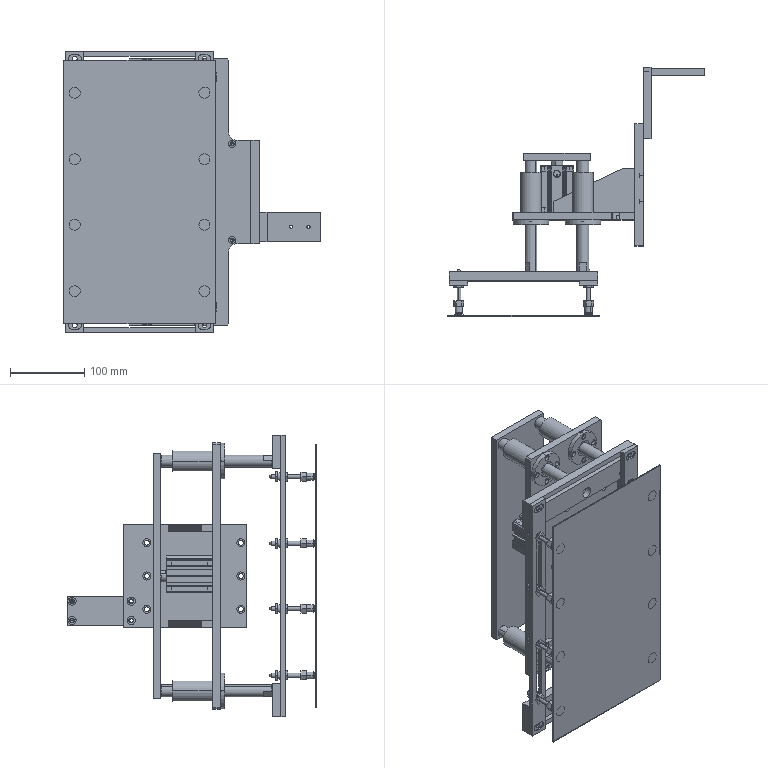Assembly | SolidWorks | mm | 30 component files | 30 solids | 1263 faces | box 346.5 x 335.9 x 380 mm | volume 1913881 mm3 | cylinder 546 | plane 505 | cone 168 | torus 32 | spline 12 | commonest cylinder face diameters 10 x40 0.4 x36 3.3 x32 4.5 x32 7.5 x32 6 x32 11 x28 6.6 x28
Bill of materials:
SL021-102-4065.SL4PRT | 4 | Bearing Steel | Long, slender cylindrical rod with a small axial hole at one end and a short flat on the outside next to that end.
SL021-102-4066.SL4PRT | 1 | AL6061 | Flat rectangular plate of even thickness with many round through holes spread around its edges and in the interior.
SL021-102-4067.SL4PRT | 2 | AL6061 | Flat plate of even thickness with a trapezoid outline (one sloped edge), with holes drilled into its narrow side edges.
SL021-102-4073.SL4PRT | 1 | AL6061 | Rectangular block or thick plate with four round through holes near its corners. The two holes at one end look larger than the two at the other.
SL021-102-4074.SL4PRT | 1 | AL6061 | Rectangular block with two small round through holes in a row on one large face, set off-center toward one end.
SL021-102-4096.SL4PRT | 1 | AL6061 | Long rectangular bar with one long slot with rounded ends running along one edge, and two round through holes near the opposite edge, toward one end.
SL021-102-4097.SL4PRT | 1 | AL6061 | Long rectangular bar with one long slot with rounded ends near one long edge, and two round through holes near the opposite edge, toward one end.
SL021-102-4098.SL4PRT | 2 | AL6061 | Thin, long, narrow strip with two long slots with rounded ends along its center line and a small round hole near each end.
SL021-102-4099.SL4PRT | 1 | AL6061 | Flat plate shaped like a rectangle with a tab sticking out from one long side. Rounded notches sit where the tab meets the plate. Four large round holes, each ringed by four small holes, are near the corners, with more small holes in the middle and on the tab.
SL021-102-4100.SL4PRT | 1 | AL6061 | Thin flat rectangular plate with four small round holes near the corners and one small hole in the center.
SL021-113Q32x30S (1)-2.sl4prt | 1 |  | Stepped round pin: a large-diameter head with grooves around it and a wider collar, then a smaller straight shaft with a short flat near its free end.
SL021-113Q32x30S (2)-2.sl4prt | 1 |  | Prism-shaped body made by extruding a near-square cross-section, with a large central round bore, four smaller holes running the full length near the corners, and slots running lengthwise on its sides. One side has a raised pad with two round holes.
SL021-1LGP-15.6.SL4PRT | 1 | AL6061 | Flat rectangular plate or sheet with no visible thickness and no holes or other features.
SL021-1RoundFlangeExtendedType-416.SL4PRT | 4 | Q235 | Flanged cylindrical sleeve: a long round tube with a round flange at one end. The flange has four evenly spaced holes around a central through-bore.
SL021-1SuctionCup.SL4PRT | 8 | AL6061 | Stepped round shaft with a wide flared, conical head at one end and a chamfered tip at the other. Three hexagonal features sit along the shaft.
Mates:
1. coincident | SL021-102-4097.SL4PRT-1 face at (-136.163, -102.499, 16.122) dir (0, -1, 0) | SL021-102-4098.SL4PRT-5 face at (-223.663, -102.499, -151.378) dir (0, 1, 0)
2. coincident | SL021-102-4098.SL4PRT-5 face at (-223.663, -102.499, -151.378) dir (0, 1, 0) | SL021-102-4098.SL4PRT-6 face at (-48.663, -102.499, -151.378) dir (0, 1, 0)
3. coincident | SL021-102-4098.SL4PRT-5 face at (-236.163, -102.499, 38.622) dir (0, 0, 1) | SL021-102-4098.SL4PRT-6 face at (-61.163, -102.499, 38.622) dir (0, 0, 1)
4. coincident | SL021-102-4097.SL4PRT-1 face at (-36.163, -90.499, 38.622) dir (1, 0, 0) | SL021-102-4096.SL4PRT-1 face at (-36.163, -102.499, -341.378) dir (1, 0, 0)
5. coincident | SL021-102-4065.SL4PRT-5 face at (-126.163, 59.501, -306.378) dir (0, 1, 0) | SL021-102-4100.SL4PRT-1 face at (-91.163, 59.501, -151.378) dir (0, -1, 0)
6. concentric | SL021-102-4065.SL4PRT-5 face at (-126.163, 59.501, -306.378) dir (0, -1, 0) r 8 | SL021-102-4099.SL4PRT-1 face at (-126.163, -10.499, -306.378) dir (0, -1, 0) r 14.05
7. coincident | SL021-102-4099.SL4PRT-1 face at (-83.663, -10.499, -151.378) dir (0, 1, 0) | SL021-113Q32x30S-2.SL41SM-1/SL021-113Q32x30S (2)-2.sl4prt-1 face at (-91.163, -10.499, -151.378) dir (0, -1, 0)
8. width | SL021-102-4099.SL4PRT-1 face at (-16.163, -20.499, -331.378) dir (0, 0, -1) | SL021-102-4099.SL4PRT-1 face at (-16.163, -20.499, 28.622) dir (0, 0, 1) | SL021-113Q32x30S-2.SL41SM-1/SL021-113Q32x30S (2)-2.sl4prt-1 face at (-104.663, 52.501, -173.878) dir (0, 0, -1) | SL021-113Q32x30S-2.SL41SM-1/SL021-113Q32x30S (2)-2.sl4prt-1 face at (-111.663, 52.501, -128.878) dir (0, 0, 1)
9. coincident | SL021-102-4100.SL4PRT-1 face at (-91.163, 59.501, -151.378) dir (0, -1, 0) | SL021-113Q32x30S-2.SL41SM-1/SL021-113Q32x30S (1)-2.sl4prt-1 face at (-88.197, 59.501, -148.885) dir (0, 1, 0)
10. coincident | SL021-102-4098.SL4PRT-6 face at (-48.663, -108.499, -151.378) dir (0, -1, 0) | SL021-1SuctionCup.SL4PRT-1 face at (-48.663, -108.499, -17.378) dir (0, 1, 0)
11. concentric | SL021-102-4098.SL4PRT-6 face at (-48.663, -108.499, -17.378) dir (0, 1, 0) r 5.25 | SL021-1SuctionCup.SL4PRT-1 face at (-48.663, -129.499, -17.378) dir (0, 1, 0) r 3
12. coincident | SL021-1SuctionCup.SL4PRT-1 face at (-48.663, -149.499, -17.378) dir (0, -1, 0) | SL021-1SuctionCup.SL4PRT-2 face at (-223.663, -149.499, -17.378) dir (0, -1, 0)
13. coincident | SL021-1SuctionCup.SL4PRT-2 face at (-223.663, -149.499, -17.378) dir (0, -1, 0) | SL021-1SuctionCup.SL4PRT-3 face at (-48.663, -149.499, -285.378) dir (0, -1, 0)
14. coincident | SL021-1SuctionCup.SL4PRT-3 face at (-48.663, -149.499, -285.378) dir (0, -1, 0) | SL021-1SuctionCup.SL4PRT-4 face at (-223.663, -149.499, -285.378) dir (0, -1, 0)
15. coincident | SL021-1SuctionCup.SL4PRT-4 face at (-223.663, -149.499, -285.378) dir (0, -1, 0) | SL021-1SuctionCup.SL4PRT-5 face at (-48.663, -149.499, -195.378) dir (0, -1, 0)
16. coincident | SL021-1SuctionCup.SL4PRT-5 face at (-48.663, -149.499, -195.378) dir (0, -1, 0) | SL021-1SuctionCup.SL4PRT-6 face at (-48.663, -149.499, -107.378) dir (0, -1, 0)
17. coincident | SL021-1SuctionCup.SL4PRT-6 face at (-48.663, -149.499, -107.378) dir (0, -1, 0) | SL021-1SuctionCup.SL4PRT-7 face at (-223.663, -149.499, -107.378) dir (0, -1, 0)
18. coincident | SL021-1SuctionCup.SL4PRT-7 face at (-223.663, -149.499, -107.378) dir (0, -1, 0) | SL021-1SuctionCup.SL4PRT-8 face at (-223.663, -149.499, -195.378) dir (0, -1, 0)
19. concentric | SL021-102-4098.SL4PRT-5 face at (-223.663, -108.499, -17.378) dir (0, 1, 0) r 5.25 | SL021-1SuctionCup.SL4PRT-2 face at (-223.663, -98.499, -17.378) dir (0, -1, 0) r 5
20. concentric | SL021-102-4098.SL4PRT-6 face at (-48.663, -108.499, -285.378) dir (0, 1, 0) r 5.25 | SL021-1SuctionCup.SL4PRT-3 face at (-48.663, -129.499, -285.378) dir (0, 1, 0) r 3
21. concentric | SL021-102-4098.SL4PRT-5 face at (-223.663, -108.499, -285.378) dir (0, 1, 0) r 5.25 | SL021-1SuctionCup.SL4PRT-4 face at (-223.663, -129.499, -285.378) dir (0, 1, 0) r 3
22. concentric | SL021-102-4098.SL4PRT-6 face at (-48.663, -108.499, -195.378) dir (0, 1, 0) r 5.25 | SL021-1SuctionCup.SL4PRT-5 face at (-48.663, -129.499, -195.378) dir (0, 1, 0) r 3
23. concentric | SL021-102-4098.SL4PRT-6 face at (-48.663, -108.499, -107.378) dir (0, 1, 0) r 5.25 | SL021-1SuctionCup.SL4PRT-6 face at (-48.663, -129.499, -107.378) dir (0, 1, 0) r 3
24. concentric | SL021-102-4098.SL4PRT-5 face at (-223.663, -108.499, -107.378) dir (0, 1, 0) r 5.25 | SL021-1SuctionCup.SL4PRT-7 face at (-223.663, -87.499, -107.378) dir (0, -1, 0) r 3
25. concentric | SL021-102-4098.SL4PRT-5 face at (-223.663, -108.499, -195.378) dir (0, 1, 0) r 5.25 | SL021-1SuctionCup.SL4PRT-8 face at (-223.663, -129.499, -195.378) dir (0, 1, 0) r 3
26. coincident | SL021-102-4099.SL4PRT-1 face at (13.837, -20.499, -81.378) dir (0, 0, 1) | SL021-102-4066.SL4PRT-1 face at (25.837, -55.499, -81.378) dir (0, 0, 1)
27. coincident | SL021-102-4067.SL4PRT-1 face at (13.837, 49.501, -91.378) dir (0, 1, 0) | SL021-102-4067.SL4PRT-2 face at (13.837, 49.501, -221.378) dir (0, 1, 0)
28. coincident | SL021-102-4067.SL4PRT-1 face at (13.837, -10.499, -91.378) dir (1, 0, 0) | SL021-102-4067.SL4PRT-2 face at (13.837, -10.499, -221.378) dir (1, 0, 0)
29. coincident | SL021-102-4099.SL4PRT-1 face at (-83.663, -10.499, -151.378) dir (0, 1, 0) | SL021-102-4067.SL4PRT-1 face at (-96.163, -10.499, -91.378) dir (0, -1, 0)
30. coincident | SL021-102-4066.SL4PRT-1 face at (13.837, 27.001, -151.378) dir (-1, 0, 0) | SL021-102-4067.SL4PRT-1 face at (13.837, -10.499, -91.378) dir (1, 0, 0)
31. coincident | SL021-102-4066.SL4PRT-1 face at (25.837, -55.499, -81.378) dir (0, 0, 1) | SL021-102-4067.SL4PRT-1 face at (13.837, -10.499, -81.378) dir (0, 0, 1)
32. coincident | SL021-102-4066.SL4PRT-1 face at (25.837, -55.499, -221.378) dir (0, 0, -1) | SL021-102-4067.SL4PRT-2 face at (13.837, -10.499, -221.378) dir (0, 0, -1)
33. coincident | SL021-102-4073.SL4PRT-1 face at (35.837, 137.501, -198.378) dir (1, 0, 0) | SL021-102-4074.SL4PRT-1 face at (35.837, 184.501, -218.378) dir (-1, 0, 0)
34. concentric | SL021-102-4073.SL4PRT-1 face at (25.837, 179.501, -185.378) dir (-1, 0, 0) r 5.5 | SL021-102-4074.SL4PRT-1 face at (35.837, 179.501, -185.378) dir (-1, 0, 0) r 2.5
35. parallel | SL021-102-4073.SL4PRT-1 face at (25.837, 185.501, -218.378) dir (0, 1, 0) | SL021-102-4074.SL4PRT-1 face at (71.837, 184.501, -198.378) dir (0, 1, 0)
36. coincident | SL021-102-4066.SL4PRT-1 face at (25.837, 27.001, -151.378) dir (1, 0, 0) | SL021-102-4073.SL4PRT-1 face at (25.837, 137.501, -198.378) dir (-1, 0, 0)
37. concentric | SL021-102-4066.SL4PRT-1 face at (13.837, 99.501, -211.378) dir (-1, 0, 0) r 3.3 | SL021-102-4073.SL4PRT-1 face at (25.837, 99.501, -211.378) dir (-1, 0, 0) r 2.5
38. concentric | SL021-102-4066.SL4PRT-1 face at (13.837, 99.501, -185.378) dir (-1, 0, 0) r 3.3 | SL021-102-4073.SL4PRT-1 face at (25.837, 99.501, -185.378) dir (-1, 0, 0) r 2.5
39. coincident | SL021-102-4098.SL4PRT-6 face at (-36.163, -102.499, -341.378) dir (1, 0, 0) | SL021-102-4096.SL4PRT-1 face at (-36.163, -102.499, -341.378) dir (1, 0, 0)
40. coincident | SL021-102-4098.SL4PRT-5 face at (-236.163, -102.499, -341.378) dir (-1, 0, 0) | SL021-102-4096.SL4PRT-1 face at (-236.163, -102.499, -341.378) dir (-1, 0, 0)
41. concentric | SL021-102-4099.SL4PRT-1 face at (-126.163, -10.499, -306.378) dir (0, -1, 0) r 14.05 | SL021-1RoundFlangeExtendedType-416.SL4PRT-1 face at (-126.163, 43.501, -306.378) dir (0, 1, 0) r 14
42. coincident | SL021-102-4099.SL4PRT-1 face at (-83.663, -20.499, -151.378) dir (0, -1, 0) | SL021-1RoundFlangeExtendedType-416.SL4PRT-1 face at (-126.163, -20.499, -318.378) dir (0, 1, 0)
43. parallel | SL021-102-4099.SL4PRT-1 face at (-151.163, -20.499, -331.378) dir (-1, 0, 0) | SL021-1RoundFlangeExtendedType-416.SL4PRT-1 plane at (-126.163, -26.499, -306.378) dir (-1, 0, 0)
44. parallel | SL021-102-4100.SL4PRT-1 face at (-136.163, 59.501, -316.378) dir (-1, 0, 0) | SL021-102-4099.SL4PRT-1 face at (-151.163, -20.499, -331.378) dir (-1, 0, 0)
45. parallel | SL021-102-4097.SL4PRT-1 face at (-236.163, -90.499, -6.378) dir (0, 0, -1) | SL021-102-4099.SL4PRT-1 face at (-16.163, -20.499, 28.622) dir (0, 0, 1)
46. coincident | SL021-102-4097.SL4PRT-1 face at (-236.163, -90.499, 38.622) dir (0, 0, 1) | SL021-102-4098.SL4PRT-5 face at (-236.163, -102.499, 38.622) dir (0, 0, 1)
47. coincident | SL021-102-4099.SL4PRT-1 face at (-83.663, -20.499, -151.378) dir (0, -1, 0) | SL021-1RoundFlangeExtendedType-416.SL4PRT-4 face at (-56.163, -20.499, 15.622) dir (0, 1, 0)
48. coincident | SL021-102-4099.SL4PRT-1 face at (-83.663, -20.499, -151.378) dir (0, -1, 0) | SL021-1RoundFlangeExtendedType-416.SL4PRT-3 face at (-56.163, -20.499, -294.378) dir (0, 1, 0)
49. parallel | SL021-102-4099.SL4PRT-1 face at (-151.163, -20.499, -331.378) dir (-1, 0, 0) | SL021-1RoundFlangeExtendedType-416.SL4PRT-3 plane at (-56.163, -26.499, -306.378) dir (1, 0, 0)
50. parallel | SL021-102-4099.SL4PRT-1 face at (-151.163, -20.499, -331.378) dir (-1, 0, 0) | SL021-1RoundFlangeExtendedType-416.SL4PRT-4 plane at (-56.163, -26.499, 3.622) dir (1, 0, 0)
51. concentric | SL021-1RoundFlangeExtendedType-416.SL4PRT-3 face at (-56.163, 43.501, -306.378) dir (0, 1, 0) r 8 | SL021-102-4065.SL4PRT-8 face at (-56.163, 59.501, -306.378) dir (0, -1, 0) r 8
52. concentric | SL021-1RoundFlangeExtendedType-416.SL4PRT-4 face at (-56.163, 43.501, 3.622) dir (0, 1, 0) r 14 | SL021-102-4065.SL4PRT-9 face at (-56.163, 59.501, 3.622) dir (0, -1, 0) r 8
53. coincident | SL021-102-4065.SL4PRT-8 face at (-56.163, 59.501, -306.378) dir (0, 1, 0) | SL021-102-4065.SL4PRT-9 face at (-56.163, 59.501, 3.622) dir (0, 1, 0)
54. coincident | SL021-102-4100.SL4PRT-1 face at (-91.163, 59.501, -151.378) dir (0, -1, 0) | SL021-102-4065.SL4PRT-9 face at (-56.163, 59.501, 3.622) dir (0, 1, 0)
55. concentric | SL021-102-4099.SL4PRT-1 face at (-56.163, -10.499, 3.622) dir (0, -1, 0) r 14.05 | SL021-1RoundFlangeExtendedType-416.SL4PRT-4 face at (-56.163, 43.501, 3.622) dir (0, 1, 0) r 14
56. concentric | SL021-102-4099.SL4PRT-1 face at (-56.163, -10.499, -306.378) dir (0, -1, 0) r 14.05 | SL021-1RoundFlangeExtendedType-416.SL4PRT-3 face at (-56.163, 43.501, -306.378) dir (0, 1, 0) r 14
57. concentric | SL021-102-4065.SL4PRT-5 face at (-126.163, 59.501, -306.378) dir (0, -1, 0) r 8 | SL021-102-4096.SL4PRT-1 face at (-126.163, -102.499, -306.378) dir (0, -1, 0) r 7.5
58. coincident | SL021-102-4097.SL4PRT-1 face at (-136.163, -90.499, 16.122) dir (0, 1, 0) | SL021-102-4096.SL4PRT-1 face at (-136.163, -90.499, -318.878) dir (0, 1, 0)
59. coincident | SL021-102-4097.SL4PRT-1 face at (-136.163, -90.499, 16.122) dir (0, 1, 0) | SL021-102-4065.SL4PRT-5 face at (-126.163, -90.499, -306.378) dir (0, -1, 0)
60. coincident | SL021-1SuctionCup.SL4PRT-2 face at (-223.663, -149.499, -17.378) dir (0, -1, 0) | SL021-1LGP-15.6.SL4PRT-1 face at (-136.163, -149.499, -151.378) dir (0, 1, 0)
61. concentric | SL021-102-4100.SL4PRT-1 face at (-126.163, 59.501, 3.622) dir (0, -1, 0) r 4.25 | SL021-102-4065.SL4PRT-7 face at (-126.163, 59.501, 3.622) dir (0, -1, 0) r 8
62. width | SL021-102-4100.SL4PRT-1 face at (-136.163, 59.501, -316.378) dir (-1, 0, 0) | SL021-102-4100.SL4PRT-1 face at (-46.163, 59.501, -316.378) dir (1, 0, 0) | SL021-113Q32x30S-2.SL41SM-1/SL021-113Q32x30S (2)-2.sl4prt-1 face at (-113.663, 52.501, -137.878) dir (-1, 0, 0) | SL021-113Q32x30S-2.SL41SM-1/SL021-113Q32x30S (2)-2.sl4prt-1 face at (-68.663, 52.501, -130.878) dir (1, 0, 0)
63. width | SL021-102-4096.SL4PRT-1 face at (-236.163, -102.499, -341.378) dir (-1, 0, 0) | SL021-102-4096.SL4PRT-1 face at (-36.163, -102.499, -341.378) dir (1, 0, 0) | SL021-1LGP-15.6.SL4PRT-1 face at (-238.663, -149.499, -328.878) dir (-1, 0, 0) | SL021-1LGP-15.6.SL4PRT-1 face at (-33.663, -149.499, -328.878) dir (1, 0, 0)
64. width | SL021-1LGP-15.6.SL4PRT-1 face at (-238.663, -149.499, -328.878) dir (0, 0, -1) | SL021-1LGP-15.6.SL4PRT-1 face at (-238.663, -149.499, 26.122) dir (0, 0, 1) | SL021-102-4096.SL4PRT-1 face at (-236.163, -102.499, -341.378) dir (0, 0, -1) | SL021-102-4097.SL4PRT-1 face at (-236.163, -90.499, 38.622) dir (0, 0, 1)
65. width | SL021-102-4096.SL4PRT-1 face at (-236.163, -102.499, -341.378) dir (0, 0, -1) | SL021-102-4097.SL4PRT-1 face at (-236.163, -90.499, 38.622) dir (0, 0, 1) | SL021-102-4099.SL4PRT-1 face at (-16.163, -20.499, -331.378) dir (0, 0, -1) | SL021-102-4099.SL4PRT-1 face at (-16.163, -20.499, 28.622) dir (0, 0, 1)
66. coincident | SL021-102-4099.SL4PRT-1 face at (13.837, -15.499, -151.378) dir (1, 0, 0) | SL021-102-4066.SL4PRT-1 face at (13.837, 27.001, -151.378) dir (-1, 0, 0)
67. distance | SL021-102-4099.SL4PRT-1 face at (-83.663, -20.499, -151.378) dir (0, -1, 0) | SL021-102-4066.SL4PRT-1 face at (25.837, 109.501, -81.378) dir (0, 1, 0)
68. concentric | SL021-113Q32x30S (1)-2.sl4prt-1 face at (-3.375, 0, 0) dir (1, 0, 0) r 8 | SL021-113Q32x30S (2)-2.sl4prt-1 face at (34.5, 0, 0) dir (1, 0, 0) r 16
69. distance | SL021-113Q32x30S (1)-2.sl4prt-1 face at (58.5, 6.46, -2.946) dir (1, 0, 0) | SL021-113Q32x30S (2)-2.sl4prt-1 face at (58.5, 0, 8) dir (-1, 0, 0)